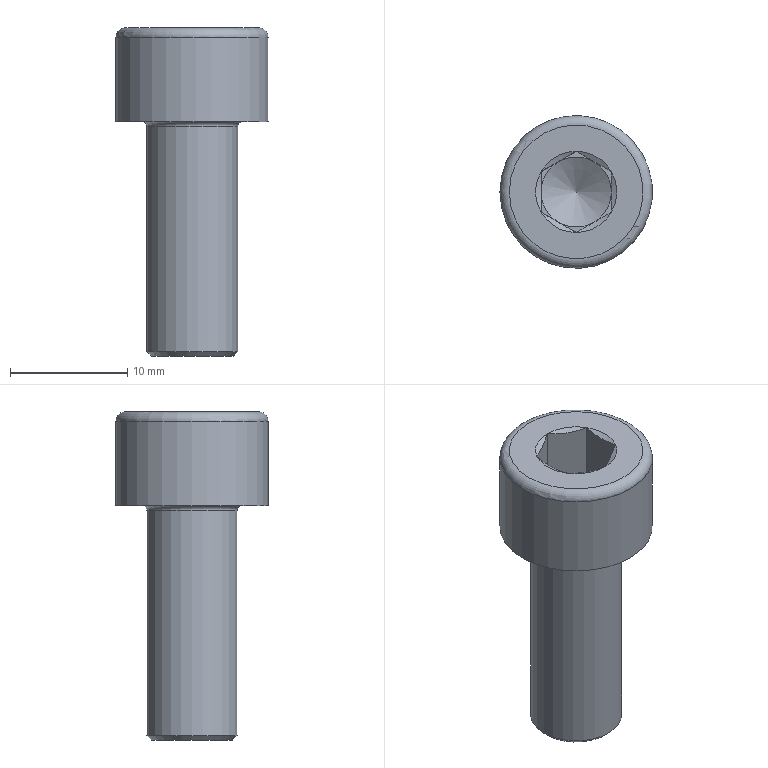Component | NX | GB-T70_1-2000_M8X20_2 | 1 solid | 27 faces | volume 1837 mm3 | plane 15 | cone 8 | cylinder 2 | torus 2 | commonest cylinder face diameters 7.76 x1 13 x1